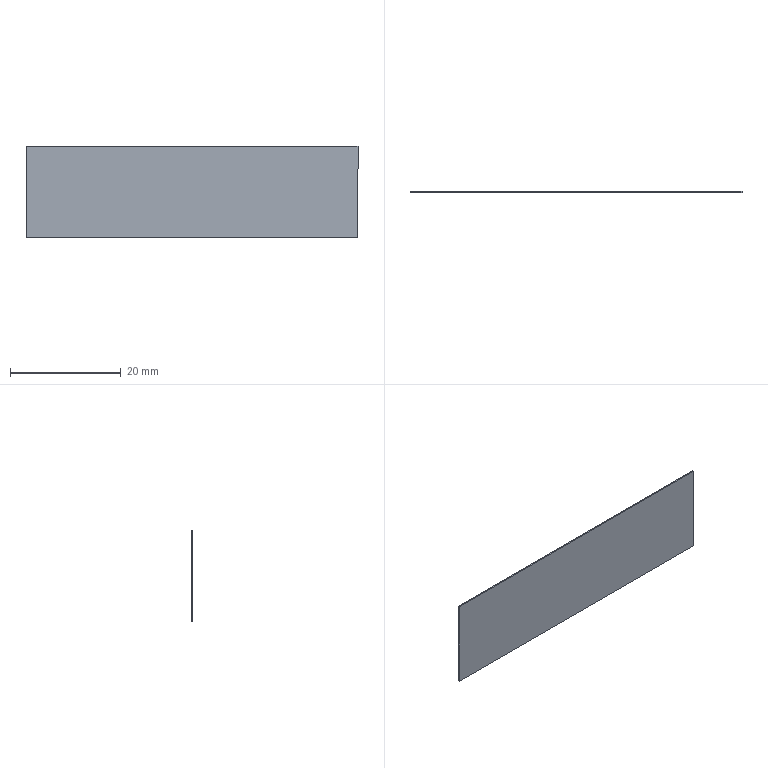Component | SolidWorks | AdapterAluminumSheetCellAssembly-1_AdapterAluminumPlate-1 | 1 solid | 11 faces | box 60 x 0.21 x 16.5 mm | volume 199 mm3 | plane 11 | material 6061
build123d program:
from build123d import *

# Parameters (mm, degrees)
SKETCH1_W           = 60
SKETCH1_H           = 16.5
BOSS_EXTRUDE1_DEPTH = 0.2
SKETCH2_W           = 30
SKETCH2_H           = 3
BOSS_EXTRUDE2_DEPTH = 0.01


with BuildPart() as part:
    # Sketch1 → Boss-Extrude1 (new body)
    with BuildSketch(Plane(origin=(0, 0, 0), x_dir=(1, 0, 0), z_dir=(0, 1, 0))):
        Rectangle(SKETCH1_W, SKETCH1_H)
    extrude(amount=BOSS_EXTRUDE1_DEPTH)

    # Sketch2 → Boss-Extrude2 (add)
    with BuildSketch(Plane(origin=(0, 0.2, 0), x_dir=(1, 0, 0), z_dir=(0, 1, 0))):
        with Locations((0, -5.25)):
            Rectangle(SKETCH2_W, SKETCH2_H)
    extrude(amount=BOSS_EXTRUDE2_DEPTH)


solid = part.part

# Placed as in the assembly
solid = solid.moved(Location((-22.49, 4.213, 36.658), (180, 0, 0)))
STEP:
#1=COLOUR_RGB('',0.7922,0.8196,0.9333);
#2=FILL_AREA_STYLE_COLOUR('',#1);
#3=FILL_AREA_STYLE('',(#2));
#4=SURFACE_STYLE_FILL_AREA(#3);
#5=SURFACE_SIDE_STYLE('',(#4));
#6=SURFACE_STYLE_USAGE(.BOTH.,#5);
#7=PRESENTATION_STYLE_ASSIGNMENT((#6));
#8=CARTESIAN_POINT('',(0.2957,0.1658,1.768));
#9=VERTEX_POINT('',#8);
#10=CARTESIAN_POINT('',(0.2957,0.1658,1.118));
#11=VERTEX_POINT('',#10);
#12=CARTESIAN_POINT('',(0.2957,0.1658,1.118));
#13=DIRECTION('',(-0.,0.,-1.));
#14=VECTOR('',#13,39.37);
#15=LINE('',#12,#14);
#16=EDGE_CURVE('',#9,#11,#15,.T.);
#17=ORIENTED_EDGE('',*,*,#16,.T.);
#18=CARTESIAN_POINT('',(-2.067,0.1658,1.118));
#19=VERTEX_POINT('',#18);
#20=CARTESIAN_POINT('',(0.2957,0.1658,1.118));
#21=DIRECTION('',(-1.,0.,0.));
#22=VECTOR('',#21,39.37);
#23=LINE('',#20,#22);
#24=EDGE_CURVE('',#11,#19,#23,.T.);
#25=ORIENTED_EDGE('',*,*,#24,.T.);
#26=CARTESIAN_POINT('',(-2.067,0.1658,1.768));
#27=VERTEX_POINT('',#26);
#28=CARTESIAN_POINT('',(-2.067,0.1658,1.118));
#29=DIRECTION('',(0.,-0.,1.));
#30=VECTOR('',#29,39.37);
#31=LINE('',#28,#30);
#32=EDGE_CURVE('',#19,#27,#31,.T.);
#33=ORIENTED_EDGE('',*,*,#32,.T.);
#34=CARTESIAN_POINT('',(0.2957,0.1658,1.768));
#35=DIRECTION('',(1.,-0.,-0.));
#36=VECTOR('',#35,39.37);
#37=LINE('',#34,#36);
#38=EDGE_CURVE('',#27,#9,#37,.T.);
#39=ORIENTED_EDGE('',*,*,#38,.T.);
#40=EDGE_LOOP('',(#17,#25,#33,#39));
#41=FACE_OUTER_BOUND('',#40,.T.);
#42=CARTESIAN_POINT('',(-0.2949,0.1658,1.296));
#43=VERTEX_POINT('',#42);
#44=CARTESIAN_POINT('',(-0.2949,0.1658,1.177));
#45=VERTEX_POINT('',#44);
#46=CARTESIAN_POINT('',(-0.2949,0.1658,1.296));
#47=DIRECTION('',(-0.,0.,-1.));
#48=VECTOR('',#47,39.37);
#49=LINE('',#46,#48);
#50=EDGE_CURVE('',#43,#45,#49,.T.);
#51=ORIENTED_EDGE('',*,*,#50,.F.);
#52=CARTESIAN_POINT('',(-1.476,0.1658,1.296));
#53=VERTEX_POINT('',#52);
#54=CARTESIAN_POINT('',(-0.2949,0.1658,1.296));
#55=DIRECTION('',(1.,-0.,-0.));
#56=VECTOR('',#55,39.37);
#57=LINE('',#54,#56);
#58=EDGE_CURVE('',#53,#43,#57,.T.);
#59=ORIENTED_EDGE('',*,*,#58,.F.);
#60=CARTESIAN_POINT('',(-1.476,0.1658,1.177));
#61=VERTEX_POINT('',#60);
#62=CARTESIAN_POINT('',(-1.476,0.1658,1.296));
#63=DIRECTION('',(0.,-0.,1.));
#64=VECTOR('',#63,39.37);
#65=LINE('',#62,#64);
#66=EDGE_CURVE('',#61,#53,#65,.T.);
#67=ORIENTED_EDGE('',*,*,#66,.F.);
#68=CARTESIAN_POINT('',(-0.2949,0.1658,1.177));
#69=DIRECTION('',(-1.,0.,0.));
#70=VECTOR('',#69,39.37);
#71=LINE('',#68,#70);
#72=EDGE_CURVE('',#45,#61,#71,.T.);
#73=ORIENTED_EDGE('',*,*,#72,.F.);
#74=EDGE_LOOP('',(#51,#59,#67,#73));
#75=FACE_BOUND('',#74,.T.);
#76=CARTESIAN_POINT('',(-0.8854,0.1658,1.443));
#77=DIRECTION('',(-0.,-1.,-0.));
#78=DIRECTION('',(0.,-0.,1.));
#79=AXIS2_PLACEMENT_3D('',#76,#77,#78);
#80=PLANE('',#79);
#81=ADVANCED_FACE('',(#41,#75),#80,.F.);
#82=CARTESIAN_POINT('',(0.2957,0.158,1.768));
#83=VERTEX_POINT('',#82);
#84=CARTESIAN_POINT('',(0.2957,0.158,1.118));
#85=VERTEX_POINT('',#84);
#86=CARTESIAN_POINT('',(0.2957,0.158,1.118));
#87=DIRECTION('',(-0.,0.,-1.));
#88=VECTOR('',#87,39.37);
#89=LINE('',#86,#88);
#90=EDGE_CURVE('',#83,#85,#89,.T.);
#91=ORIENTED_EDGE('',*,*,#90,.T.);
#92=CARTESIAN_POINT('',(0.2957,0.1658,1.118));
#93=DIRECTION('',(-0.,-1.,-0.));
#94=VECTOR('',#93,39.37);
#95=LINE('',#92,#94);
#96=EDGE_CURVE('',#11,#85,#95,.T.);
#97=ORIENTED_EDGE('',*,*,#96,.F.);
#98=ORIENTED_EDGE('',*,*,#16,.F.);
#99=CARTESIAN_POINT('',(0.2957,0.1658,1.768));
#100=DIRECTION('',(-0.,-1.,-0.));
#101=VECTOR('',#100,39.37);
#102=LINE('',#99,#101);
#103=EDGE_CURVE('',#9,#83,#102,.T.);
#104=ORIENTED_EDGE('',*,*,#103,.T.);
#105=EDGE_LOOP('',(#91,#97,#98,#104));
#106=FACE_OUTER_BOUND('',#105,.T.);
#107=CARTESIAN_POINT('',(0.2957,0.1658,1.118));
#108=DIRECTION('',(-1.,0.,0.));
#109=DIRECTION('',(0.,-0.,1.));
#110=AXIS2_PLACEMENT_3D('',#107,#108,#109);
#111=PLANE('',#110);
#112=ADVANCED_FACE('',(#106),#111,.F.);
#113=CARTESIAN_POINT('',(-2.067,0.158,1.118));
#114=VERTEX_POINT('',#113);
#115=CARTESIAN_POINT('',(0.2957,0.158,1.118));
#116=DIRECTION('',(-1.,0.,0.));
#117=VECTOR('',#116,39.37);
#118=LINE('',#115,#117);
#119=EDGE_CURVE('',#85,#114,#118,.T.);
#120=ORIENTED_EDGE('',*,*,#119,.T.);
#121=CARTESIAN_POINT('',(-2.067,0.1658,1.118));
#122=DIRECTION('',(-0.,-1.,-0.));
#123=VECTOR('',#122,39.37);
#124=LINE('',#121,#123);
#125=EDGE_CURVE('',#19,#114,#124,.T.);
#126=ORIENTED_EDGE('',*,*,#125,.F.);
#127=ORIENTED_EDGE('',*,*,#24,.F.);
#128=ORIENTED_EDGE('',*,*,#96,.T.);
#129=EDGE_LOOP('',(#120,#126,#127,#128));
#130=FACE_OUTER_BOUND('',#129,.T.);
#131=CARTESIAN_POINT('',(0.2957,0.1658,1.118));
#132=DIRECTION('',(0.,-0.,1.));
#133=DIRECTION('',(1.,-0.,-0.));
#134=AXIS2_PLACEMENT_3D('',#131,#132,#133);
#135=PLANE('',#134);
#136=ADVANCED_FACE('',(#130),#135,.F.);
#137=CARTESIAN_POINT('',(-2.067,0.158,1.768));
#138=VERTEX_POINT('',#137);
#139=CARTESIAN_POINT('',(-2.067,0.158,1.118));
#140=DIRECTION('',(0.,-0.,1.));
#141=VECTOR('',#140,39.37);
#142=LINE('',#139,#141);
#143=EDGE_CURVE('',#114,#138,#142,.T.);
#144=ORIENTED_EDGE('',*,*,#143,.T.);
#145=CARTESIAN_POINT('',(-2.067,0.1658,1.768));
#146=DIRECTION('',(-0.,-1.,-0.));
#147=VECTOR('',#146,39.37);
#148=LINE('',#145,#147);
#149=EDGE_CURVE('',#27,#138,#148,.T.);
#150=ORIENTED_EDGE('',*,*,#149,.F.);
#151=ORIENTED_EDGE('',*,*,#32,.F.);
#152=ORIENTED_EDGE('',*,*,#125,.T.);
#153=EDGE_LOOP('',(#144,#150,#151,#152));
#154=FACE_OUTER_BOUND('',#153,.T.);
#155=CARTESIAN_POINT('',(-2.067,0.1658,1.118));
#156=DIRECTION('',(1.,-0.,-0.));
#157=DIRECTION('',(-0.,0.,-1.));
#158=AXIS2_PLACEMENT_3D('',#155,#156,#157);
#159=PLANE('',#158);
#160=ADVANCED_FACE('',(#154),#159,.F.);
#161=CARTESIAN_POINT('',(0.2957,0.158,1.768));
#162=DIRECTION('',(1.,-0.,-0.));
#163=VECTOR('',#162,39.37);
#164=LINE('',#161,#163);
#165=EDGE_CURVE('',#138,#83,#164,.T.);
#166=ORIENTED_EDGE('',*,*,#165,.T.);
#167=ORIENTED_EDGE('',*,*,#103,.F.);
#168=ORIENTED_EDGE('',*,*,#38,.F.);
#169=ORIENTED_EDGE('',*,*,#149,.T.);
#170=EDGE_LOOP('',(#166,#167,#168,#169));
#171=FACE_OUTER_BOUND('',#170,.T.);
#172=CARTESIAN_POINT('',(0.2957,0.1658,1.768));
#173=DIRECTION('',(-0.,0.,-1.));
#174=DIRECTION('',(-1.,0.,0.));
#175=AXIS2_PLACEMENT_3D('',#172,#173,#174);
#176=PLANE('',#175);
#177=ADVANCED_FACE('',(#171),#176,.F.);
#178=ORIENTED_EDGE('',*,*,#90,.F.);
#179=ORIENTED_EDGE('',*,*,#165,.F.);
#180=ORIENTED_EDGE('',*,*,#143,.F.);
#181=ORIENTED_EDGE('',*,*,#119,.F.);
#182=EDGE_LOOP('',(#178,#179,#180,#181));
#183=FACE_OUTER_BOUND('',#182,.T.);
#184=CARTESIAN_POINT('',(-0.8854,0.158,1.443));
#185=DIRECTION('',(-0.,-1.,-0.));
#186=DIRECTION('',(0.,-0.,1.));
#187=AXIS2_PLACEMENT_3D('',#184,#185,#186);
#188=PLANE('',#187);
#189=ADVANCED_FACE('',(#183),#188,.T.);
#190=ORIENTED_EDGE('',*,*,#50,.T.);
#191=CARTESIAN_POINT('',(-0.2949,0.1662,1.177));
#192=VERTEX_POINT('',#191);
#193=CARTESIAN_POINT('',(-0.2949,0.1662,1.177));
#194=DIRECTION('',(-0.,-1.,-0.));
#195=VECTOR('',#194,39.37);
#196=LINE('',#193,#195);
#197=EDGE_CURVE('',#192,#45,#196,.T.);
#198=ORIENTED_EDGE('',*,*,#197,.F.);
#199=CARTESIAN_POINT('',(-0.2949,0.1662,1.296));
#200=VERTEX_POINT('',#199);
#201=CARTESIAN_POINT('',(-0.2949,0.1662,1.296));
#202=DIRECTION('',(-0.,0.,-1.));
#203=VECTOR('',#202,39.37);
#204=LINE('',#201,#203);
#205=EDGE_CURVE('',#200,#192,#204,.T.);
#206=ORIENTED_EDGE('',*,*,#205,.F.);
#207=CARTESIAN_POINT('',(-0.2949,0.1662,1.296));
#208=DIRECTION('',(-0.,-1.,-0.));
#209=VECTOR('',#208,39.37);
#210=LINE('',#207,#209);
#211=EDGE_CURVE('',#200,#43,#210,.T.);
#212=ORIENTED_EDGE('',*,*,#211,.T.);
#213=EDGE_LOOP('',(#190,#198,#206,#212));
#214=FACE_OUTER_BOUND('',#213,.T.);
#215=CARTESIAN_POINT('',(-0.2949,0.1662,1.296));
#216=DIRECTION('',(-1.,0.,0.));
#217=DIRECTION('',(0.,-0.,1.));
#218=AXIS2_PLACEMENT_3D('',#215,#216,#217);
#219=PLANE('',#218);
#220=ADVANCED_FACE('',(#214),#219,.F.);
#221=ORIENTED_EDGE('',*,*,#72,.T.);
#222=CARTESIAN_POINT('',(-1.476,0.1662,1.177));
#223=VERTEX_POINT('',#222);
#224=CARTESIAN_POINT('',(-1.476,0.1662,1.177));
#225=DIRECTION('',(-0.,-1.,-0.));
#226=VECTOR('',#225,39.37);
#227=LINE('',#224,#226);
#228=EDGE_CURVE('',#223,#61,#227,.T.);
#229=ORIENTED_EDGE('',*,*,#228,.F.);
#230=CARTESIAN_POINT('',(-0.2949,0.1662,1.177));
#231=DIRECTION('',(-1.,0.,0.));
#232=VECTOR('',#231,39.37);
#233=LINE('',#230,#232);
#234=EDGE_CURVE('',#192,#223,#233,.T.);
#235=ORIENTED_EDGE('',*,*,#234,.F.);
#236=ORIENTED_EDGE('',*,*,#197,.T.);
#237=EDGE_LOOP('',(#221,#229,#235,#236));
#238=FACE_OUTER_BOUND('',#237,.T.);
#239=CARTESIAN_POINT('',(-0.2949,0.1662,1.177));
#240=DIRECTION('',(0.,-0.,1.));
#241=DIRECTION('',(1.,-0.,-0.));
#242=AXIS2_PLACEMENT_3D('',#239,#240,#241);
#243=PLANE('',#242);
#244=ADVANCED_FACE('',(#238),#243,.F.);
#245=ORIENTED_EDGE('',*,*,#66,.T.);
#246=CARTESIAN_POINT('',(-1.476,0.1662,1.296));
#247=VERTEX_POINT('',#246);
#248=CARTESIAN_POINT('',(-1.476,0.1662,1.296));
#249=DIRECTION('',(-0.,-1.,-0.));
#250=VECTOR('',#249,39.37);
#251=LINE('',#248,#250);
#252=EDGE_CURVE('',#247,#53,#251,.T.);
#253=ORIENTED_EDGE('',*,*,#252,.F.);
#254=CARTESIAN_POINT('',(-1.476,0.1662,1.296));
#255=DIRECTION('',(0.,-0.,1.));
#256=VECTOR('',#255,39.37);
#257=LINE('',#254,#256);
#258=EDGE_CURVE('',#223,#247,#257,.T.);
#259=ORIENTED_EDGE('',*,*,#258,.F.);
#260=ORIENTED_EDGE('',*,*,#228,.T.);
#261=EDGE_LOOP('',(#245,#253,#259,#260));
#262=FACE_OUTER_BOUND('',#261,.T.);
#263=CARTESIAN_POINT('',(-1.476,0.1662,1.296));
#264=DIRECTION('',(1.,-0.,-0.));
#265=DIRECTION('',(-0.,0.,-1.));
#266=AXIS2_PLACEMENT_3D('',#263,#264,#265);
#267=PLANE('',#266);
#268=ADVANCED_FACE('',(#262),#267,.F.);
#269=ORIENTED_EDGE('',*,*,#58,.T.);
#270=ORIENTED_EDGE('',*,*,#211,.F.);
#271=CARTESIAN_POINT('',(-0.2949,0.1662,1.296));
#272=DIRECTION('',(1.,-0.,-0.));
#273=VECTOR('',#272,39.37);
#274=LINE('',#271,#273);
#275=EDGE_CURVE('',#247,#200,#274,.T.);
#276=ORIENTED_EDGE('',*,*,#275,.F.);
#277=ORIENTED_EDGE('',*,*,#252,.T.);
#278=EDGE_LOOP('',(#269,#270,#276,#277));
#279=FACE_OUTER_BOUND('',#278,.T.);
#280=CARTESIAN_POINT('',(-0.2949,0.1662,1.296));
#281=DIRECTION('',(-0.,0.,-1.));
#282=DIRECTION('',(-1.,0.,0.));
#283=AXIS2_PLACEMENT_3D('',#280,#281,#282);
#284=PLANE('',#283);
#285=ADVANCED_FACE('',(#279),#284,.F.);
#286=ORIENTED_EDGE('',*,*,#205,.T.);
#287=ORIENTED_EDGE('',*,*,#234,.T.);
#288=ORIENTED_EDGE('',*,*,#258,.T.);
#289=ORIENTED_EDGE('',*,*,#275,.T.);
#290=EDGE_LOOP('',(#286,#287,#288,#289));
#291=FACE_OUTER_BOUND('',#290,.T.);
#292=CARTESIAN_POINT('',(-0.8854,0.1662,1.443));
#293=DIRECTION('',(0.,1.,0.));
#294=DIRECTION('',(-0.,0.,-1.));
#295=AXIS2_PLACEMENT_3D('',#292,#293,#294);
#296=PLANE('',#295);
#297=ADVANCED_FACE('',(#291),#296,.T.);
#298=CLOSED_SHELL('',(#81,#112,#136,#160,#177,#189,#220,#244,#268,#285,#297));
#299=MANIFOLD_SOLID_BREP('',#298);
#300=STYLED_ITEM('',(#7),#299);
#301=PRESENTATION_LAYER_ASSIGNMENT('','',(#300));
#302=CARTESIAN_POINT('',(0.,0.,0.));
#303=DIRECTION('',(0.,0.,1.));
#304=DIRECTION('',(1.,0.,0.));
#305=AXIS2_PLACEMENT_3D('',#302,#303,#304);
#306=(LENGTH_UNIT()NAMED_UNIT(*)SI_UNIT($,.METRE.));
#307=LENGTH_MEASURE_WITH_UNIT(LENGTH_MEASURE(0.0254),#306);
#308=DIMENSIONAL_EXPONENTS(1.,0.,0.,0.,0.,0.,0.);
#309=(CONVERSION_BASED_UNIT('',#307)LENGTH_UNIT()NAMED_UNIT(#308));
#310=UNCERTAINTY_MEASURE_WITH_UNIT(LENGTH_MEASURE(0.00001),#309,'','');
#311=(NAMED_UNIT(*)PLANE_ANGLE_UNIT()SI_UNIT($,.RADIAN.));
#312=(NAMED_UNIT(*)SI_UNIT($,.STERADIAN.)SOLID_ANGLE_UNIT());
#313=(GEOMETRIC_REPRESENTATION_CONTEXT(3)GLOBAL_UNCERTAINTY_ASSIGNED_CONTEXT((#310))GLOBAL_UNIT_ASSIGNED_CONTEXT((#309,#311,#312))REPRESENTATION_CONTEXT('',''));
#314=ADVANCED_BREP_SHAPE_REPRESENTATION('',(#299,#305),#313);
#315=(LENGTH_UNIT()NAMED_UNIT(*)SI_UNIT($,.METRE.));
#316=LENGTH_MEASURE_WITH_UNIT(LENGTH_MEASURE(0.0254),#315);
#317=DIMENSIONAL_EXPONENTS(1.,0.,0.,0.,0.,0.,0.);
#318=(CONVERSION_BASED_UNIT('',#316)LENGTH_UNIT()NAMED_UNIT(#317));
#319=UNCERTAINTY_MEASURE_WITH_UNIT(LENGTH_MEASURE(0.00001),#318,'','');
#320=(NAMED_UNIT(*)PLANE_ANGLE_UNIT()SI_UNIT($,.RADIAN.));
#321=(NAMED_UNIT(*)SI_UNIT($,.STERADIAN.)SOLID_ANGLE_UNIT());
#322=(GEOMETRIC_REPRESENTATION_CONTEXT(3)GLOBAL_UNCERTAINTY_ASSIGNED_CONTEXT((#319))GLOBAL_UNIT_ASSIGNED_CONTEXT((#318,#320,#321))REPRESENTATION_CONTEXT('',''));
#323=MECHANICAL_DESIGN_GEOMETRIC_PRESENTATION_REPRESENTATION('',(#300),#322);